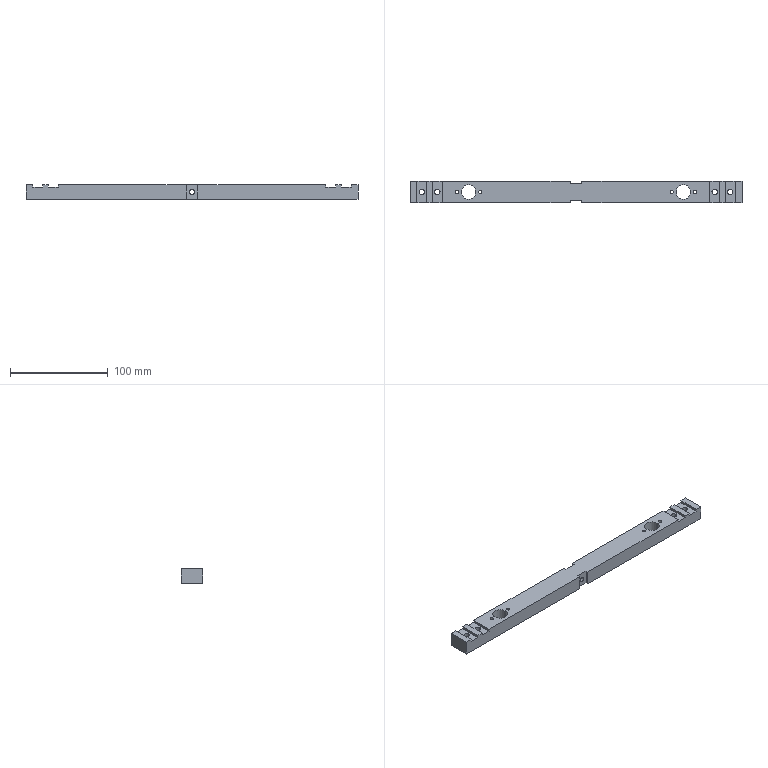Component | SolidWorks | FixedRod-1 | 1 solid | 64 faces | box 340 x 22 x 15 mm | volume 100515 mm3 | plane 34 | cylinder 30 | commonest cylinder face diameters 3.3 x8 10 x8 5.5 x8 15 x4 5 x2
build123d program:
from build123d import *

# Parameters (mm, degrees)
SKETCH1_W                                         = 340
SKETCH1_H                                         = 22
BOSS_EXTRUDE1_DEPTH                               = 15
SKETCH2_W                                         = 10
SKETCH2_H                                         = 22
CUT_EXTRUDE1_DEPTH                                = 2.5
HOLE_SIZE_ACCORDING_TO_HEXAGON_SOCKET_D           = 5.5
HOLE_SIZE_ACCORDING_TO_HEXAGON_SOCKET_DEPTH       = 15.2
HOLE_SIZE_ACCORDING_TO_HEXAGON_SOCKET_CBORE_D     = 10
HOLE_SIZE_ACCORDING_TO_HEXAGON_SOCKET_CBORE_DEPTH = 5.7
HOLE_SIZE_ACCORDING_TO_HEXAGON_SOCKET_TIP         = 1.652
F_15_0_15_DIAMETER_HOLE1_D                        = 15
SKETCH7_R                                         = 2.5
CUT_EXTRUDE2_DEPTH                                = 342.041
SKETCH9_W                                         = 12
SKETCH9_H                                         = 15
CUT_EXTRUDE3_DEPTH                                = 2.5
M4_TAPPED_HOLE1_D                                 = 3.3


with BuildPart() as part:
    # Sketch1 → Boss-Extrude1 (new body)
    with BuildSketch(Plane.XY):
        with Locations((170, 11)):
            Rectangle(SKETCH1_W, SKETCH1_H)
    extrude(amount=BOSS_EXTRUDE1_DEPTH)

    # Sketch2 → Cut-Extrude1 (cut)
    with BuildSketch(Plane.XY.offset(15)):
        with Locations((12, 11)):
            Rectangle(SKETCH2_W, SKETCH2_H)
        with Locations((28, 11)):
            Rectangle(SKETCH2_W, SKETCH2_H)
        with Locations((328, 11)):
            Rectangle(SKETCH2_W, SKETCH2_H)
        with Locations((312, 11)):
            Rectangle(SKETCH2_W, SKETCH2_H)
    extrude(amount=-CUT_EXTRUDE1_DEPTH, mode=Mode.SUBTRACT)

    # Hole Size _According to_ Hexagon Socket
    with Locations(Plane(origin=(328, 11, 0), x_dir=(-1, 0, 0), z_dir=(0, 0, -1))):
        with Locations((0, 0), (16, 0), (316, 0), (300, 0)):
            CounterBoreHole(HOLE_SIZE_ACCORDING_TO_HEXAGON_SOCKET_D / 2, HOLE_SIZE_ACCORDING_TO_HEXAGON_SOCKET_CBORE_D / 2, HOLE_SIZE_ACCORDING_TO_HEXAGON_SOCKET_CBORE_DEPTH, depth=HOLE_SIZE_ACCORDING_TO_HEXAGON_SOCKET_DEPTH)
            with Locations((0, 0, -(HOLE_SIZE_ACCORDING_TO_HEXAGON_SOCKET_DEPTH + HOLE_SIZE_ACCORDING_TO_HEXAGON_SOCKET_TIP / 2))):  # 118° drill point
                Cone(0, HOLE_SIZE_ACCORDING_TO_HEXAGON_SOCKET_D / 2, HOLE_SIZE_ACCORDING_TO_HEXAGON_SOCKET_TIP, mode=Mode.SUBTRACT)

    # 15.0 _15_ Diameter Hole1 (through all)
    with Locations(Plane(origin=(60, 11, 0), x_dir=(-1, 0, 0), z_dir=(0, 0, -1))):
        with Locations((0, 0), (-220, 0)):
            Hole(F_15_0_15_DIAMETER_HOLE1_D / 2)

    # Sketch7 → Cut-Extrude2 (cut, through all)
    with BuildSketch(Plane.XZ):
        with Locations(Location((170, 7.5, 0), (0, 0, 270))):
            Circle(SKETCH7_R)
    extrude(amount=-CUT_EXTRUDE2_DEPTH, mode=Mode.SUBTRACT)

    # Sketch9 → Cut-Extrude3 (cut)
    with BuildSketch(Plane.XZ):
        with Locations((170, 7.5)):
            Rectangle(SKETCH9_W, SKETCH9_H)
    cut_extrude3 = extrude(amount=-CUT_EXTRUDE3_DEPTH, mode=Mode.SUBTRACT)

    # Mirror1: Cut-Extrude3 across plane
    add(cut_extrude3.mirror(Plane(origin=(0, 11, 0), x_dir=(0, 0, 1), z_dir=(0, -1, 0))), mode=Mode.SUBTRACT)

    # M4 Tapped Hole1 (through all)
    with Locations(Plane(origin=(48, 11, 15), x_dir=(1, 0, 0), z_dir=(0, 0, 1))):
        with Locations((0, 0), (24, 0), (220, 0), (244, 0)):
            Hole(M4_TAPPED_HOLE1_D / 2)


solid = part.part

# Placed as in the assembly
solid = solid.moved(Location((-30, -230.228, 56), (0, 0, 0)))